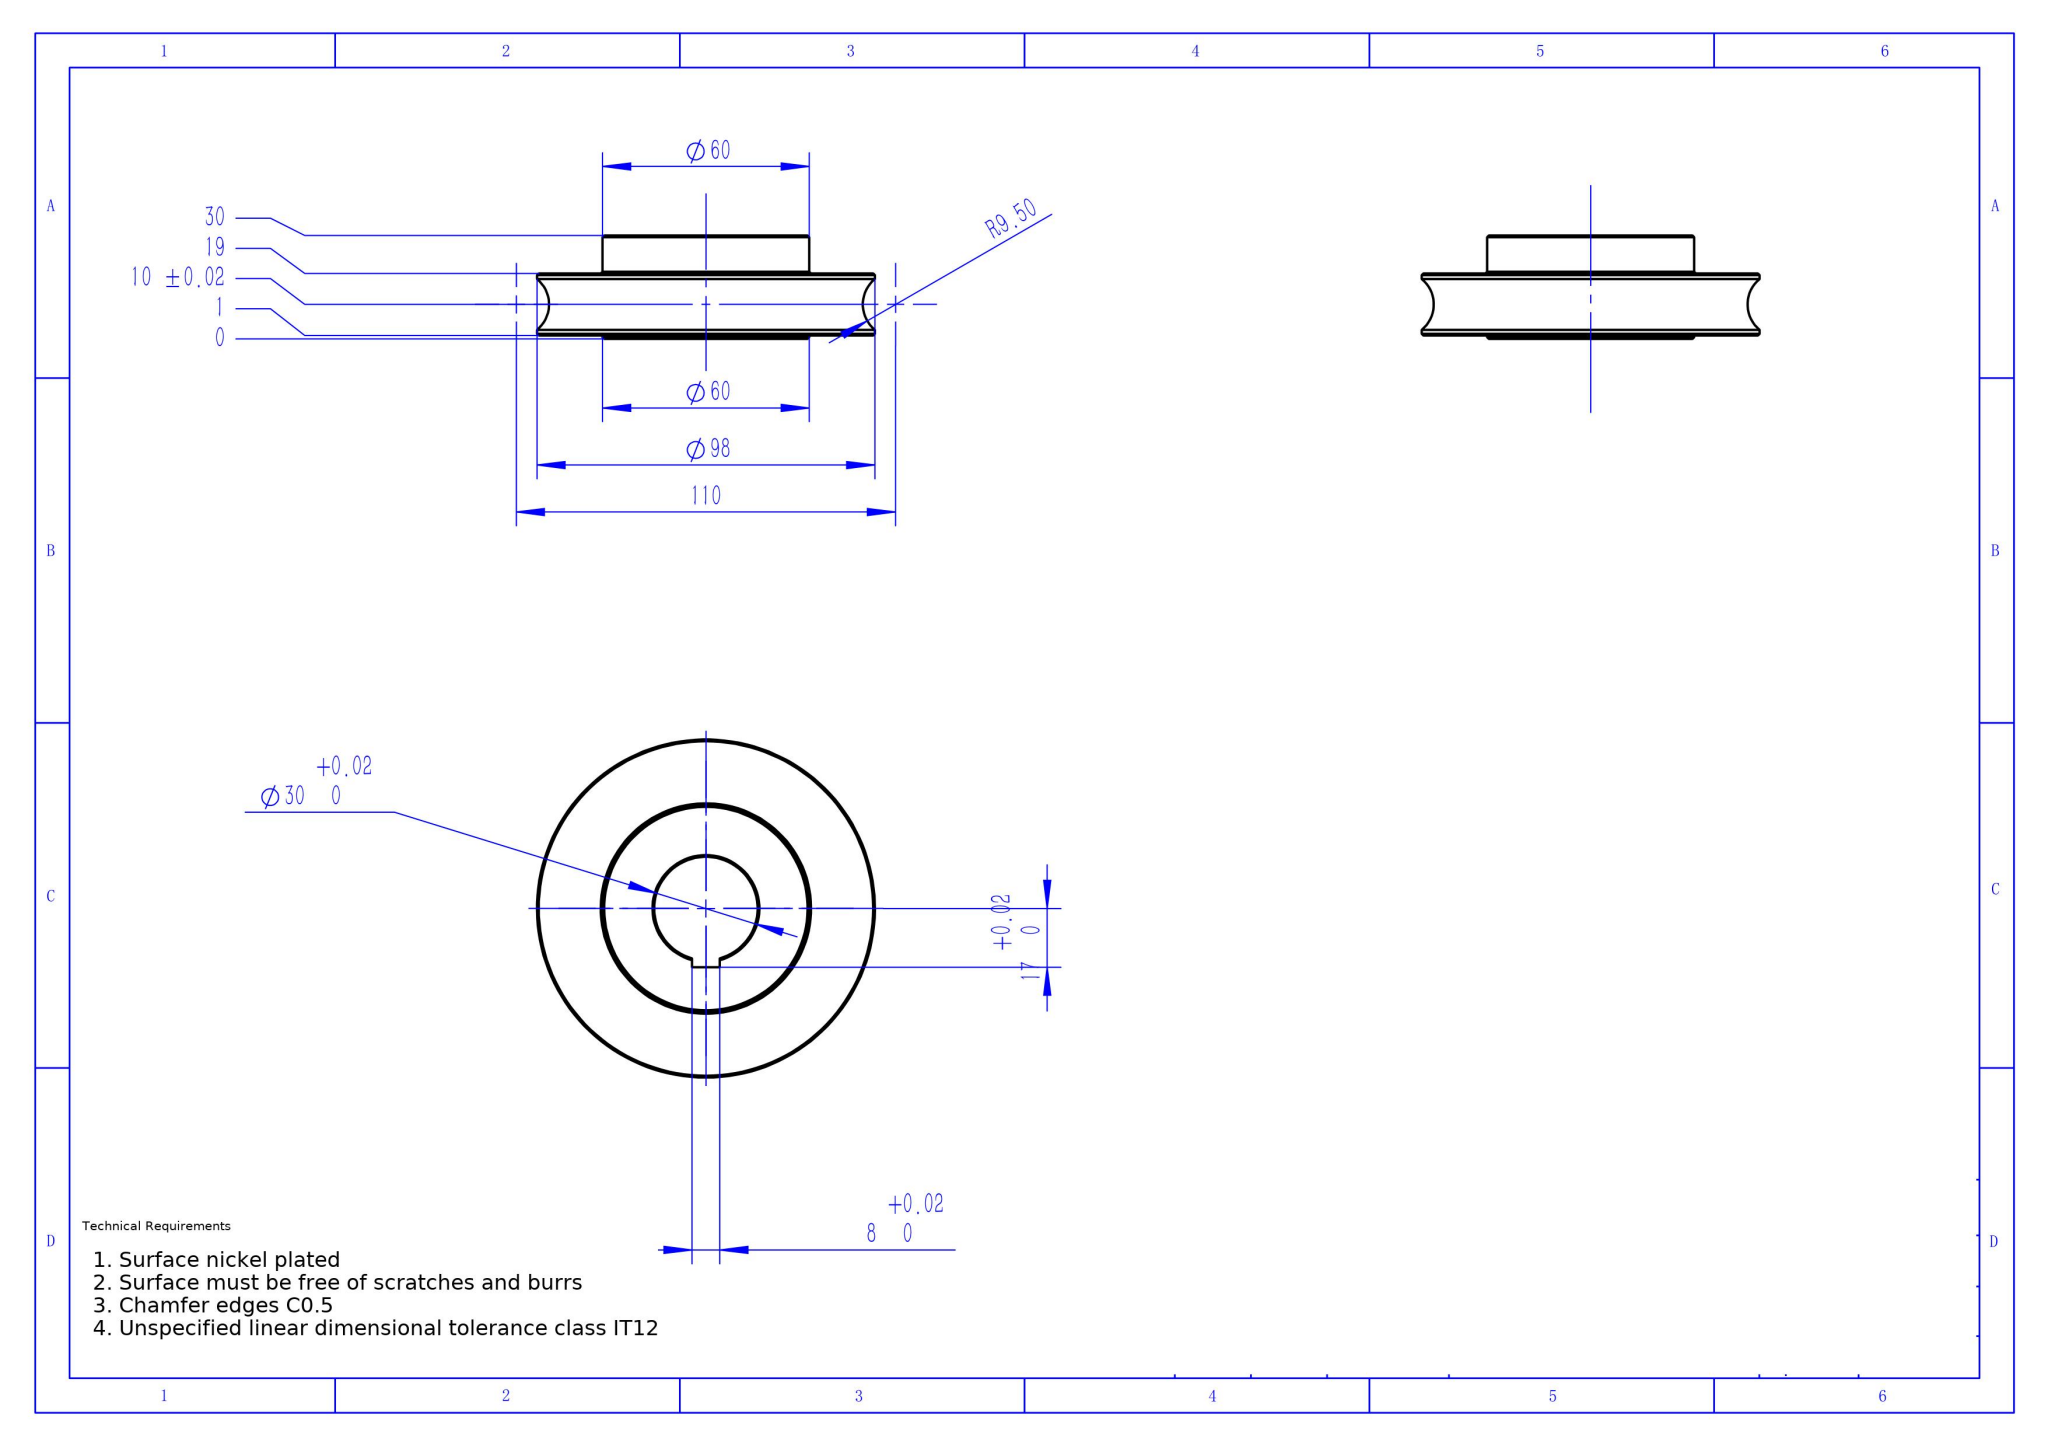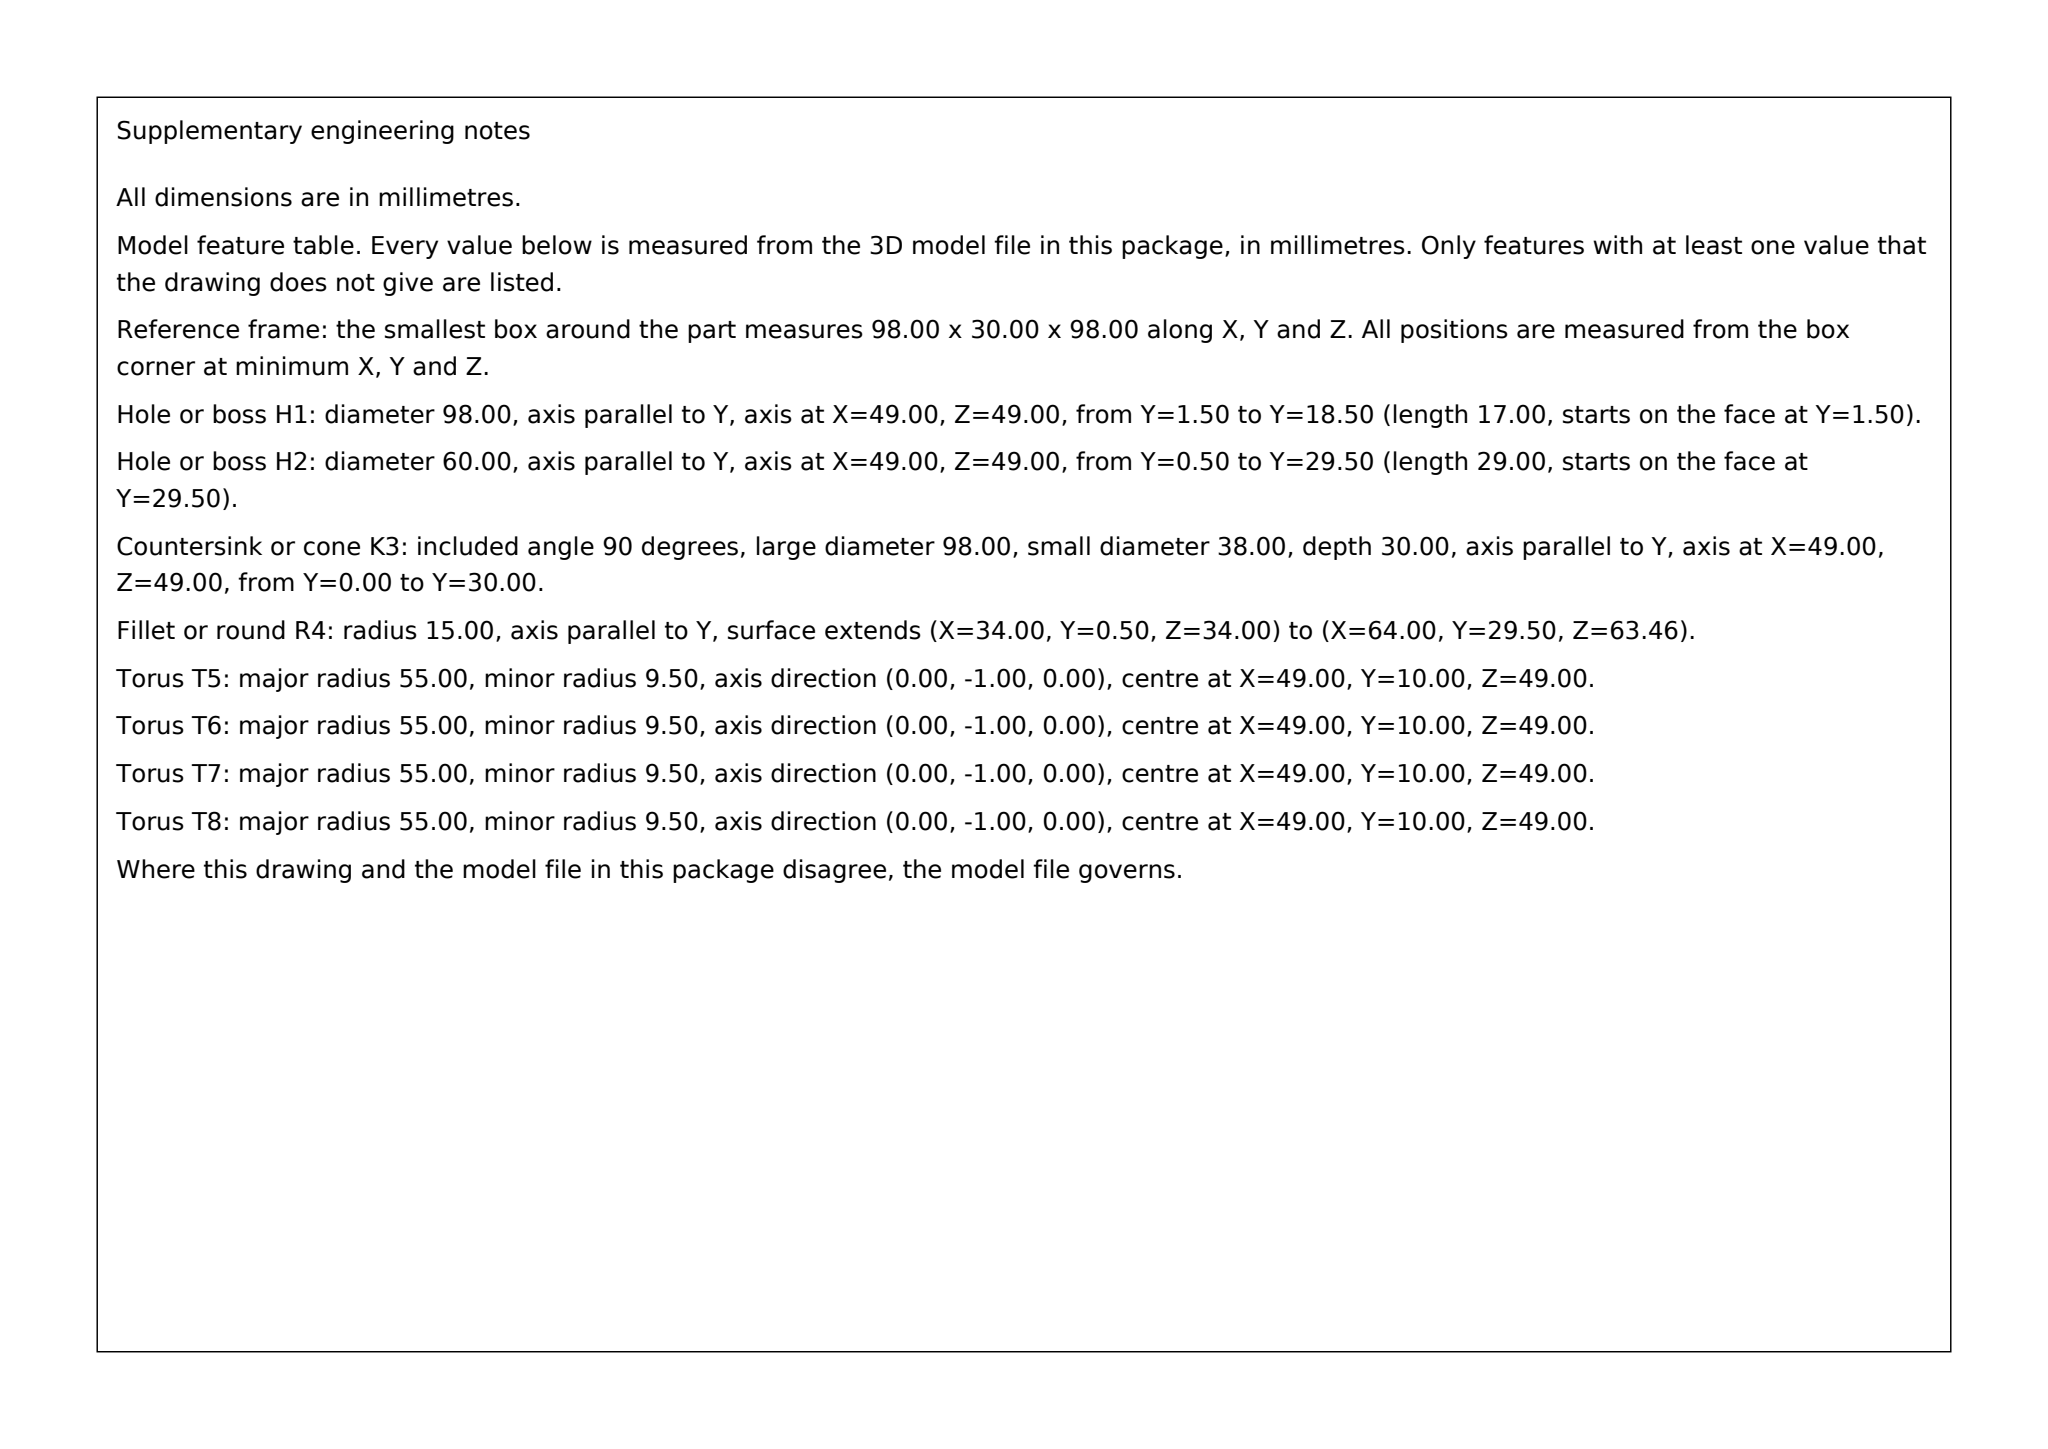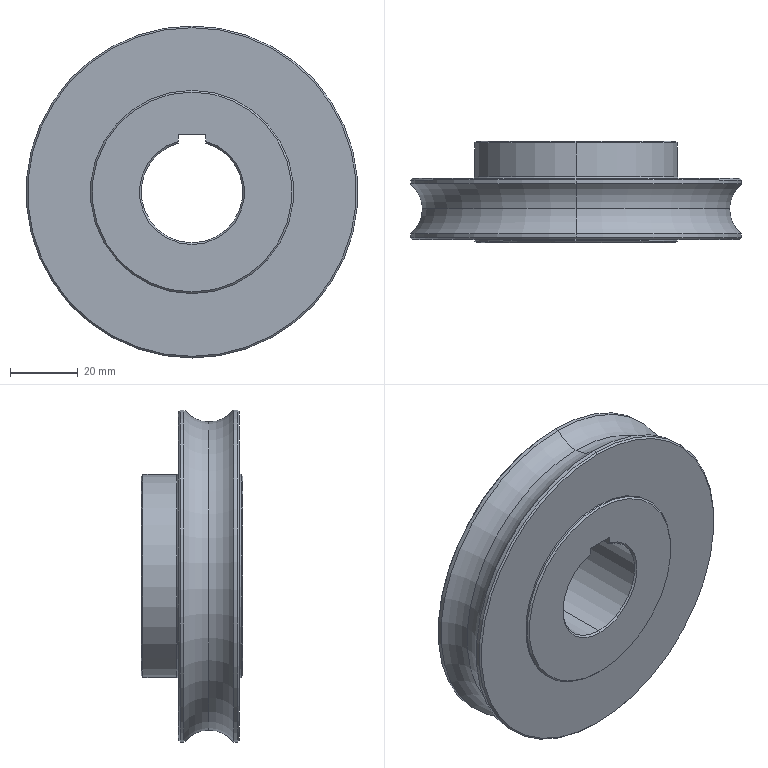Part | SolidWorks | mm | 1 solid | 34 faces | box 98 x 30 x 98 mm | volume 137127 mm3 | cone 13 | cylinder 10 | plane 7 | torus 4 | commonest cylinder face diameters 60 x4 98 x4 30 x2
build123d program:
from build123d import *

# Parameters (mm, degrees)
CHAMFER1_SIZE              = 0.5
KEYWAY_DEPTH               = 95.362
F_16_0_16_DIAMETER_HOLE1_D = 16


with BuildPart() as part:
    # Sketch1 → Revolve1 (revolve)
    with BuildSketch(Plane.XY, mode=Mode.PRIVATE) as revolve1_sk:
        with BuildLine():
            Line((15, -10), (15, 20))
            Line((15, 20), (30, 20))
            Line((30, 20), (30, 9))
            Line((30, 9), (49, 9))
            Line((49, 9), (49, 7.365))
            ThreePointArc((49, 7.365), (45.5, 0), (49, -7.365))
            Line((49, -7.365), (49, -9))
            Line((49, -9), (30, -9))
            Line((30, -9), (30, -10))
            Line((30, -10), (15, -10))
        make_face()
    revolve(revolve1_sk.sketch.rotate(Axis((0, 0, 0), (0, 1, 0)), 90), axis=Axis((0, 0, 0), (0, 1, 0)))

    # Chamfer1
    chamfer1_edges = [part.edges().sort_by_distance(p)[0] for p in [
        (0, -9, 49),
        (0, -10, 30),
        (0, -10, 15),
        (0, 20, 15),
        (0, 20, 30),
        (0, 9, 30),
        (0, 9, 49),
    ]]
    chamfer(chamfer1_edges, length=CHAMFER1_SIZE)

    # KeySketch → Keyway (cut, through all)
    with BuildSketch(Plane(origin=(17.778, 20, -10.539), x_dir=(-1, 0, 0), z_dir=(0, 1, 0))):
        with BuildLine():
            Line((13.778, 24.996), (13.778, 27.539))
            Line((13.778, 27.539), (21.778, 27.539))
            Line((21.778, 27.539), (21.778, 24.996))
            ThreePointArc((21.778, 24.996), (17.778, -4.461), (13.778, 24.996))
        make_face()
    extrude(amount=-KEYWAY_DEPTH, mode=Mode.SUBTRACT)

    # 16.0 _16_ Diameter Hole1 (through all)
    with Locations(Plane(origin=(0, 9, 0), x_dir=(1, 0, 0), z_dir=(0, 1, 0))):
        with Locations((-40.305, 40.305), (40.305, -40.305), (40.305, 40.305), (-40.305, -40.305)):
            Hole(F_16_0_16_DIAMETER_HOLE1_D / 2)


solid = part.part